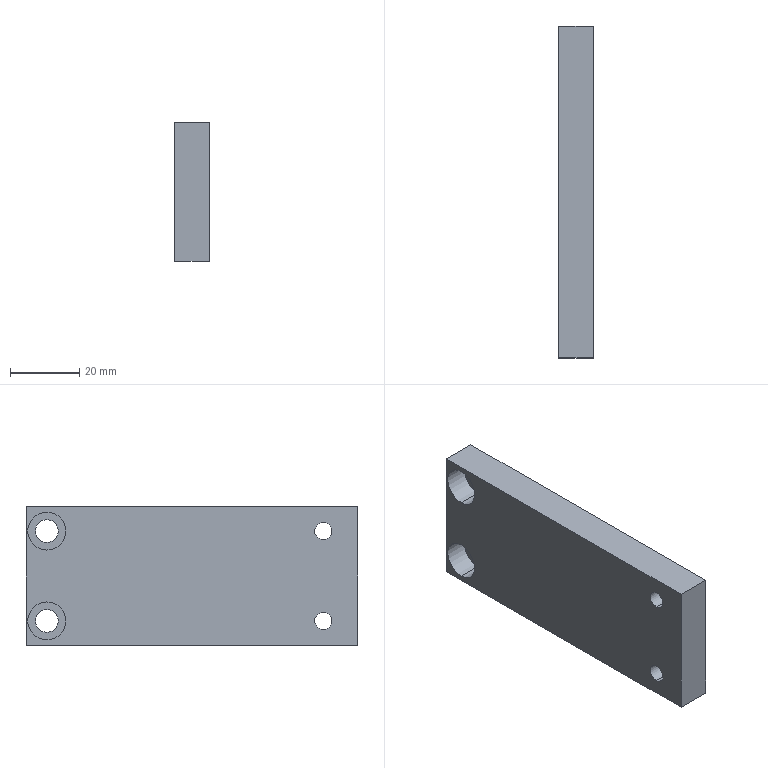Component | SolidWorks | SL021-102-4073.SL4PRT-1 | 1 solid | 20 faces | box 10 x 96 x 40 mm | volume 36496 mm3 | cylinder 12 | plane 8 | commonest cylinder face diameters 11 x4 6.6 x4 5 x4 | material AL6061
build123d program:
from build123d import *

# Parameters (mm, degrees)
SKETCH1_W                                          = 40
SKETCH1_H                                          = 96
BOSS_EXTRUDE1_DEPTH                                = 5
M6_TAPPED_HOLE1_D                                  = 5
HOLE_SIZE_ACCORDING_TO_TYPE_1_OF_HEXAG_D           = 6.6
HOLE_SIZE_ACCORDING_TO_TYPE_1_OF_HEXAG_CBORE_D     = 11
HOLE_SIZE_ACCORDING_TO_TYPE_1_OF_HEXAG_CBORE_DEPTH = 6.8


with BuildPart() as part:
    # Sketch1 → Boss-Extrude1 (new, symmetric)
    with BuildSketch(Plane.XY):
        Rectangle(SKETCH1_W, SKETCH1_H)
    extrude(amount=BOSS_EXTRUDE1_DEPTH, both=True)

    # M6 Tapped Hole1 (through all)
    with Locations(Plane.XY.offset(5)):
        with Locations((-13, -38), (13, -38)):
            Hole(M6_TAPPED_HOLE1_D / 2)

    # Hole Size _According to_ Type 1 of Hexag (through all)
    with Locations(Plane.XY.offset(5)):
        with Locations((-13, 42), (13, 42)):
            CounterBoreHole(HOLE_SIZE_ACCORDING_TO_TYPE_1_OF_HEXAG_D / 2, HOLE_SIZE_ACCORDING_TO_TYPE_1_OF_HEXAG_CBORE_D / 2, HOLE_SIZE_ACCORDING_TO_TYPE_1_OF_HEXAG_CBORE_DEPTH)


solid = part.part

# Placed as in the assembly
solid = solid.moved(Location((30.837, 137.501, -198.378), (0, -90, 0)))
STEP:
#1=COLOUR_RGB('',0.7922,0.8196,0.9333);
#2=FILL_AREA_STYLE_COLOUR('',#1);
#3=FILL_AREA_STYLE('',(#2));
#4=SURFACE_STYLE_FILL_AREA(#3);
#5=SURFACE_SIDE_STYLE('',(#4));
#6=SURFACE_STYLE_USAGE(.BOTH.,#5);
#7=PRESENTATION_STYLE_ASSIGNMENT((#6));
#8=CARTESIAN_POINT('',(1.285,7.067,-8.539));
#9=VERTEX_POINT('',#8);
#10=CARTESIAN_POINT('',(1.285,7.067,-8.105));
#11=VERTEX_POINT('',#10);
#12=CARTESIAN_POINT('',(1.285,7.067,-8.322));
#13=DIRECTION('',(-1.,0.,-0.));
#14=DIRECTION('',(0.,0.,1.));
#15=AXIS2_PLACEMENT_3D('',#12,#13,#14);
#16=CIRCLE('',#15,0.2165);
#17=EDGE_CURVE('',#9,#11,#16,.T.);
#18=ORIENTED_EDGE('',*,*,#17,.F.);
#19=CARTESIAN_POINT('',(1.017,7.067,-8.539));
#20=VERTEX_POINT('',#19);
#21=CARTESIAN_POINT('',(1.017,7.067,-8.539));
#22=DIRECTION('',(-1.,0.,-0.));
#23=VECTOR('',#22,39.37);
#24=LINE('',#21,#23);
#25=EDGE_CURVE('',#9,#20,#24,.T.);
#26=ORIENTED_EDGE('',*,*,#25,.T.);
#27=CARTESIAN_POINT('',(1.017,7.067,-8.105));
#28=VERTEX_POINT('',#27);
#29=CARTESIAN_POINT('',(1.017,7.067,-8.322));
#30=DIRECTION('',(-1.,0.,-0.));
#31=DIRECTION('',(0.,0.,1.));
#32=AXIS2_PLACEMENT_3D('',#29,#30,#31);
#33=CIRCLE('',#32,0.2165);
#34=EDGE_CURVE('',#20,#28,#33,.T.);
#35=ORIENTED_EDGE('',*,*,#34,.T.);
#36=CARTESIAN_POINT('',(1.017,7.067,-8.105));
#37=DIRECTION('',(-1.,0.,-0.));
#38=VECTOR('',#37,39.37);
#39=LINE('',#36,#38);
#40=EDGE_CURVE('',#11,#28,#39,.T.);
#41=ORIENTED_EDGE('',*,*,#40,.F.);
#42=EDGE_LOOP('',(#18,#26,#35,#41));
#43=FACE_OUTER_BOUND('',#42,.T.);
#44=CARTESIAN_POINT('',(1.017,7.067,-8.322));
#45=DIRECTION('',(-1.,0.,-0.));
#46=DIRECTION('',(0.,0.,1.));
#47=AXIS2_PLACEMENT_3D('',#44,#45,#46);
#48=CYLINDRICAL_SURFACE('',#47,0.2165);
#49=ADVANCED_FACE('',(#43),#48,.F.);
#50=CARTESIAN_POINT('',(1.411,7.067,-8.452));
#51=VERTEX_POINT('',#50);
#52=CARTESIAN_POINT('',(1.411,7.067,-8.192));
#53=VERTEX_POINT('',#52);
#54=CARTESIAN_POINT('',(1.411,7.067,-8.322));
#55=DIRECTION('',(-1.,0.,-0.));
#56=DIRECTION('',(0.,0.,1.));
#57=AXIS2_PLACEMENT_3D('',#54,#55,#56);
#58=CIRCLE('',#57,0.1299);
#59=EDGE_CURVE('',#51,#53,#58,.T.);
#60=ORIENTED_EDGE('',*,*,#59,.F.);
#61=CARTESIAN_POINT('',(1.285,7.067,-8.452));
#62=VERTEX_POINT('',#61);
#63=CARTESIAN_POINT('',(1.017,7.067,-8.452));
#64=DIRECTION('',(-1.,0.,-0.));
#65=VECTOR('',#64,39.37);
#66=LINE('',#63,#65);
#67=EDGE_CURVE('',#51,#62,#66,.T.);
#68=ORIENTED_EDGE('',*,*,#67,.T.);
#69=CARTESIAN_POINT('',(1.285,7.067,-8.192));
#70=VERTEX_POINT('',#69);
#71=CARTESIAN_POINT('',(1.285,7.067,-8.322));
#72=DIRECTION('',(-1.,0.,-0.));
#73=DIRECTION('',(0.,0.,1.));
#74=AXIS2_PLACEMENT_3D('',#71,#72,#73);
#75=CIRCLE('',#74,0.1299);
#76=EDGE_CURVE('',#62,#70,#75,.T.);
#77=ORIENTED_EDGE('',*,*,#76,.T.);
#78=CARTESIAN_POINT('',(1.017,7.067,-8.192));
#79=DIRECTION('',(-1.,0.,-0.));
#80=VECTOR('',#79,39.37);
#81=LINE('',#78,#80);
#82=EDGE_CURVE('',#53,#70,#81,.T.);
#83=ORIENTED_EDGE('',*,*,#82,.F.);
#84=EDGE_LOOP('',(#60,#68,#77,#83));
#85=FACE_OUTER_BOUND('',#84,.T.);
#86=CARTESIAN_POINT('',(1.017,7.067,-8.322));
#87=DIRECTION('',(-1.,0.,-0.));
#88=DIRECTION('',(0.,0.,1.));
#89=AXIS2_PLACEMENT_3D('',#86,#87,#88);
#90=CYLINDRICAL_SURFACE('',#89,0.1299);
#91=ADVANCED_FACE('',(#85),#90,.F.);
#92=CARTESIAN_POINT('',(1.285,7.067,-7.515));
#93=VERTEX_POINT('',#92);
#94=CARTESIAN_POINT('',(1.285,7.067,-7.082));
#95=VERTEX_POINT('',#94);
#96=CARTESIAN_POINT('',(1.285,7.067,-7.298));
#97=DIRECTION('',(-1.,0.,-0.));
#98=DIRECTION('',(0.,0.,1.));
#99=AXIS2_PLACEMENT_3D('',#96,#97,#98);
#100=CIRCLE('',#99,0.2165);
#101=EDGE_CURVE('',#93,#95,#100,.T.);
#102=ORIENTED_EDGE('',*,*,#101,.F.);
#103=CARTESIAN_POINT('',(1.017,7.067,-7.515));
#104=VERTEX_POINT('',#103);
#105=CARTESIAN_POINT('',(1.017,7.067,-7.515));
#106=DIRECTION('',(-1.,0.,-0.));
#107=VECTOR('',#106,39.37);
#108=LINE('',#105,#107);
#109=EDGE_CURVE('',#93,#104,#108,.T.);
#110=ORIENTED_EDGE('',*,*,#109,.T.);
#111=CARTESIAN_POINT('',(1.017,7.067,-7.082));
#112=VERTEX_POINT('',#111);
#113=CARTESIAN_POINT('',(1.017,7.067,-7.298));
#114=DIRECTION('',(-1.,0.,-0.));
#115=DIRECTION('',(0.,0.,1.));
#116=AXIS2_PLACEMENT_3D('',#113,#114,#115);
#117=CIRCLE('',#116,0.2165);
#118=EDGE_CURVE('',#104,#112,#117,.T.);
#119=ORIENTED_EDGE('',*,*,#118,.T.);
#120=CARTESIAN_POINT('',(1.017,7.067,-7.082));
#121=DIRECTION('',(-1.,0.,-0.));
#122=VECTOR('',#121,39.37);
#123=LINE('',#120,#122);
#124=EDGE_CURVE('',#95,#112,#123,.T.);
#125=ORIENTED_EDGE('',*,*,#124,.F.);
#126=EDGE_LOOP('',(#102,#110,#119,#125));
#127=FACE_OUTER_BOUND('',#126,.T.);
#128=CARTESIAN_POINT('',(1.017,7.067,-7.298));
#129=DIRECTION('',(-1.,0.,-0.));
#130=DIRECTION('',(0.,0.,1.));
#131=AXIS2_PLACEMENT_3D('',#128,#129,#130);
#132=CYLINDRICAL_SURFACE('',#131,0.2165);
#133=ADVANCED_FACE('',(#127),#132,.F.);
#134=CARTESIAN_POINT('',(1.411,7.067,-7.428));
#135=VERTEX_POINT('',#134);
#136=CARTESIAN_POINT('',(1.411,7.067,-7.168));
#137=VERTEX_POINT('',#136);
#138=CARTESIAN_POINT('',(1.411,7.067,-7.298));
#139=DIRECTION('',(-1.,0.,-0.));
#140=DIRECTION('',(0.,0.,1.));
#141=AXIS2_PLACEMENT_3D('',#138,#139,#140);
#142=CIRCLE('',#141,0.1299);
#143=EDGE_CURVE('',#135,#137,#142,.T.);
#144=ORIENTED_EDGE('',*,*,#143,.F.);
#145=CARTESIAN_POINT('',(1.285,7.067,-7.428));
#146=VERTEX_POINT('',#145);
#147=CARTESIAN_POINT('',(1.017,7.067,-7.428));
#148=DIRECTION('',(-1.,0.,-0.));
#149=VECTOR('',#148,39.37);
#150=LINE('',#147,#149);
#151=EDGE_CURVE('',#135,#146,#150,.T.);
#152=ORIENTED_EDGE('',*,*,#151,.T.);
#153=CARTESIAN_POINT('',(1.285,7.067,-7.168));
#154=VERTEX_POINT('',#153);
#155=CARTESIAN_POINT('',(1.285,7.067,-7.298));
#156=DIRECTION('',(-1.,0.,-0.));
#157=DIRECTION('',(0.,0.,1.));
#158=AXIS2_PLACEMENT_3D('',#155,#156,#157);
#159=CIRCLE('',#158,0.1299);
#160=EDGE_CURVE('',#146,#154,#159,.T.);
#161=ORIENTED_EDGE('',*,*,#160,.T.);
#162=CARTESIAN_POINT('',(1.017,7.067,-7.168));
#163=DIRECTION('',(-1.,0.,-0.));
#164=VECTOR('',#163,39.37);
#165=LINE('',#162,#164);
#166=EDGE_CURVE('',#137,#154,#165,.T.);
#167=ORIENTED_EDGE('',*,*,#166,.F.);
#168=EDGE_LOOP('',(#144,#152,#161,#167));
#169=FACE_OUTER_BOUND('',#168,.T.);
#170=CARTESIAN_POINT('',(1.017,7.067,-7.298));
#171=DIRECTION('',(-1.,0.,-0.));
#172=DIRECTION('',(0.,0.,1.));
#173=AXIS2_PLACEMENT_3D('',#170,#171,#172);
#174=CYLINDRICAL_SURFACE('',#173,0.1299);
#175=ADVANCED_FACE('',(#169),#174,.F.);
#176=CARTESIAN_POINT('',(1.411,3.917,-8.42));
#177=VERTEX_POINT('',#176);
#178=CARTESIAN_POINT('',(1.411,3.917,-8.224));
#179=VERTEX_POINT('',#178);
#180=CARTESIAN_POINT('',(1.411,3.917,-8.322));
#181=DIRECTION('',(-1.,0.,-0.));
#182=DIRECTION('',(0.,0.,1.));
#183=AXIS2_PLACEMENT_3D('',#180,#181,#182);
#184=CIRCLE('',#183,0.09843);
#185=EDGE_CURVE('',#177,#179,#184,.T.);
#186=ORIENTED_EDGE('',*,*,#185,.F.);
#187=CARTESIAN_POINT('',(1.017,3.917,-8.42));
#188=VERTEX_POINT('',#187);
#189=CARTESIAN_POINT('',(1.017,3.917,-8.42));
#190=DIRECTION('',(-1.,0.,-0.));
#191=VECTOR('',#190,39.37);
#192=LINE('',#189,#191);
#193=EDGE_CURVE('',#177,#188,#192,.T.);
#194=ORIENTED_EDGE('',*,*,#193,.T.);
#195=CARTESIAN_POINT('',(1.017,3.917,-8.224));
#196=VERTEX_POINT('',#195);
#197=CARTESIAN_POINT('',(1.017,3.917,-8.322));
#198=DIRECTION('',(-1.,0.,-0.));
#199=DIRECTION('',(0.,0.,1.));
#200=AXIS2_PLACEMENT_3D('',#197,#198,#199);
#201=CIRCLE('',#200,0.09843);
#202=EDGE_CURVE('',#188,#196,#201,.T.);
#203=ORIENTED_EDGE('',*,*,#202,.T.);
#204=CARTESIAN_POINT('',(1.017,3.917,-8.224));
#205=DIRECTION('',(-1.,0.,-0.));
#206=VECTOR('',#205,39.37);
#207=LINE('',#204,#206);
#208=EDGE_CURVE('',#179,#196,#207,.T.);
#209=ORIENTED_EDGE('',*,*,#208,.F.);
#210=EDGE_LOOP('',(#186,#194,#203,#209));
#211=FACE_OUTER_BOUND('',#210,.T.);
#212=CARTESIAN_POINT('',(1.017,3.917,-8.322));
#213=DIRECTION('',(-1.,0.,-0.));
#214=DIRECTION('',(0.,0.,1.));
#215=AXIS2_PLACEMENT_3D('',#212,#213,#214);
#216=CYLINDRICAL_SURFACE('',#215,0.09843);
#217=ADVANCED_FACE('',(#211),#216,.F.);
#218=CARTESIAN_POINT('',(1.411,3.917,-7.397));
#219=VERTEX_POINT('',#218);
#220=CARTESIAN_POINT('',(1.411,3.917,-7.2));
#221=VERTEX_POINT('',#220);
#222=CARTESIAN_POINT('',(1.411,3.917,-7.298));
#223=DIRECTION('',(-1.,0.,-0.));
#224=DIRECTION('',(0.,0.,1.));
#225=AXIS2_PLACEMENT_3D('',#222,#223,#224);
#226=CIRCLE('',#225,0.09843);
#227=EDGE_CURVE('',#219,#221,#226,.T.);
#228=ORIENTED_EDGE('',*,*,#227,.F.);
#229=CARTESIAN_POINT('',(1.017,3.917,-7.397));
#230=VERTEX_POINT('',#229);
#231=CARTESIAN_POINT('',(1.017,3.917,-7.397));
#232=DIRECTION('',(-1.,0.,-0.));
#233=VECTOR('',#232,39.37);
#234=LINE('',#231,#233);
#235=EDGE_CURVE('',#219,#230,#234,.T.);
#236=ORIENTED_EDGE('',*,*,#235,.T.);
#237=CARTESIAN_POINT('',(1.017,3.917,-7.2));
#238=VERTEX_POINT('',#237);
#239=CARTESIAN_POINT('',(1.017,3.917,-7.298));
#240=DIRECTION('',(-1.,0.,-0.));
#241=DIRECTION('',(0.,0.,1.));
#242=AXIS2_PLACEMENT_3D('',#239,#240,#241);
#243=CIRCLE('',#242,0.09843);
#244=EDGE_CURVE('',#230,#238,#243,.T.);
#245=ORIENTED_EDGE('',*,*,#244,.T.);
#246=CARTESIAN_POINT('',(1.017,3.917,-7.2));
#247=DIRECTION('',(-1.,0.,-0.));
#248=VECTOR('',#247,39.37);
#249=LINE('',#246,#248);
#250=EDGE_CURVE('',#221,#238,#249,.T.);
#251=ORIENTED_EDGE('',*,*,#250,.F.);
#252=EDGE_LOOP('',(#228,#236,#245,#251));
#253=FACE_OUTER_BOUND('',#252,.T.);
#254=CARTESIAN_POINT('',(1.017,3.917,-7.298));
#255=DIRECTION('',(-1.,0.,-0.));
#256=DIRECTION('',(0.,0.,1.));
#257=AXIS2_PLACEMENT_3D('',#254,#255,#256);
#258=CYLINDRICAL_SURFACE('',#257,0.09843);
#259=ADVANCED_FACE('',(#253),#258,.F.);
#260=CARTESIAN_POINT('',(1.411,7.067,-8.322));
#261=DIRECTION('',(-1.,0.,-0.));
#262=DIRECTION('',(0.,0.,1.));
#263=AXIS2_PLACEMENT_3D('',#260,#261,#262);
#264=CIRCLE('',#263,0.1299);
#265=EDGE_CURVE('',#53,#51,#264,.T.);
#266=ORIENTED_EDGE('',*,*,#265,.T.);
#267=ORIENTED_EDGE('',*,*,#59,.T.);
#268=EDGE_LOOP('',(#266,#267));
#269=FACE_BOUND('',#268,.T.);
#270=CARTESIAN_POINT('',(1.411,7.067,-7.298));
#271=DIRECTION('',(-1.,0.,-0.));
#272=DIRECTION('',(0.,0.,1.));
#273=AXIS2_PLACEMENT_3D('',#270,#271,#272);
#274=CIRCLE('',#273,0.1299);
#275=EDGE_CURVE('',#137,#135,#274,.T.);
#276=ORIENTED_EDGE('',*,*,#275,.T.);
#277=ORIENTED_EDGE('',*,*,#143,.T.);
#278=EDGE_LOOP('',(#276,#277));
#279=FACE_BOUND('',#278,.T.);
#280=CARTESIAN_POINT('',(1.411,3.524,-7.023));
#281=VERTEX_POINT('',#280);
#282=CARTESIAN_POINT('',(1.411,7.303,-7.023));
#283=VERTEX_POINT('',#282);
#284=CARTESIAN_POINT('',(1.411,3.524,-7.023));
#285=DIRECTION('',(0.,1.,0.));
#286=VECTOR('',#285,39.37);
#287=LINE('',#284,#286);
#288=EDGE_CURVE('',#281,#283,#287,.T.);
#289=ORIENTED_EDGE('',*,*,#288,.F.);
#290=CARTESIAN_POINT('',(1.411,3.524,-8.598));
#291=VERTEX_POINT('',#290);
#292=CARTESIAN_POINT('',(1.411,3.524,-8.598));
#293=DIRECTION('',(-0.,-0.,1.));
#294=VECTOR('',#293,39.37);
#295=LINE('',#292,#294);
#296=EDGE_CURVE('',#291,#281,#295,.T.);
#297=ORIENTED_EDGE('',*,*,#296,.F.);
#298=CARTESIAN_POINT('',(1.411,7.303,-8.598));
#299=VERTEX_POINT('',#298);
#300=CARTESIAN_POINT('',(1.411,3.524,-8.598));
#301=DIRECTION('',(-0.,-1.,-0.));
#302=VECTOR('',#301,39.37);
#303=LINE('',#300,#302);
#304=EDGE_CURVE('',#299,#291,#303,.T.);
#305=ORIENTED_EDGE('',*,*,#304,.F.);
#306=CARTESIAN_POINT('',(1.411,7.303,-8.598));
#307=DIRECTION('',(0.,0.,-1.));
#308=VECTOR('',#307,39.37);
#309=LINE('',#306,#308);
#310=EDGE_CURVE('',#283,#299,#309,.T.);
#311=ORIENTED_EDGE('',*,*,#310,.F.);
#312=EDGE_LOOP('',(#289,#297,#305,#311));
#313=FACE_OUTER_BOUND('',#312,.T.);
#314=CARTESIAN_POINT('',(1.411,3.917,-7.298));
#315=DIRECTION('',(-1.,0.,-0.));
#316=DIRECTION('',(0.,0.,1.));
#317=AXIS2_PLACEMENT_3D('',#314,#315,#316);
#318=CIRCLE('',#317,0.09843);
#319=EDGE_CURVE('',#221,#219,#318,.T.);
#320=ORIENTED_EDGE('',*,*,#319,.T.);
#321=ORIENTED_EDGE('',*,*,#227,.T.);
#322=EDGE_LOOP('',(#320,#321));
#323=FACE_BOUND('',#322,.T.);
#324=CARTESIAN_POINT('',(1.411,3.917,-8.322));
#325=DIRECTION('',(-1.,0.,-0.));
#326=DIRECTION('',(0.,0.,1.));
#327=AXIS2_PLACEMENT_3D('',#324,#325,#326);
#328=CIRCLE('',#327,0.09843);
#329=EDGE_CURVE('',#179,#177,#328,.T.);
#330=ORIENTED_EDGE('',*,*,#329,.T.);
#331=ORIENTED_EDGE('',*,*,#185,.T.);
#332=EDGE_LOOP('',(#330,#331));
#333=FACE_BOUND('',#332,.T.);
#334=CARTESIAN_POINT('',(1.411,5.413,-7.81));
#335=DIRECTION('',(1.,-0.,0.));
#336=DIRECTION('',(0.,0.,-1.));
#337=AXIS2_PLACEMENT_3D('',#334,#335,#336);
#338=PLANE('',#337);
#339=ADVANCED_FACE('',(#269,#279,#313,#323,#333),#338,.T.);
#340=ORIENTED_EDGE('',*,*,#288,.T.);
#341=CARTESIAN_POINT('',(1.017,7.303,-7.023));
#342=VERTEX_POINT('',#341);
#343=CARTESIAN_POINT('',(1.017,7.303,-7.023));
#344=DIRECTION('',(1.,-0.,0.));
#345=VECTOR('',#344,39.37);
#346=LINE('',#343,#345);
#347=EDGE_CURVE('',#342,#283,#346,.T.);
#348=ORIENTED_EDGE('',*,*,#347,.F.);
#349=CARTESIAN_POINT('',(1.017,3.524,-7.023));
#350=VERTEX_POINT('',#349);
#351=CARTESIAN_POINT('',(1.017,3.524,-7.023));
#352=DIRECTION('',(0.,1.,0.));
#353=VECTOR('',#352,39.37);
#354=LINE('',#351,#353);
#355=EDGE_CURVE('',#350,#342,#354,.T.);
#356=ORIENTED_EDGE('',*,*,#355,.F.);
#357=CARTESIAN_POINT('',(1.017,3.524,-7.023));
#358=DIRECTION('',(1.,-0.,0.));
#359=VECTOR('',#358,39.37);
#360=LINE('',#357,#359);
#361=EDGE_CURVE('',#350,#281,#360,.T.);
#362=ORIENTED_EDGE('',*,*,#361,.T.);
#363=EDGE_LOOP('',(#340,#348,#356,#362));
#364=FACE_OUTER_BOUND('',#363,.T.);
#365=CARTESIAN_POINT('',(1.017,3.524,-7.023));
#366=DIRECTION('',(0.,0.,-1.));
#367=DIRECTION('',(-1.,0.,-0.));
#368=AXIS2_PLACEMENT_3D('',#365,#366,#367);
#369=PLANE('',#368);
#370=ADVANCED_FACE('',(#364),#369,.F.);
#371=ORIENTED_EDGE('',*,*,#310,.T.);
#372=CARTESIAN_POINT('',(1.017,7.303,-8.598));
#373=VERTEX_POINT('',#372);
#374=CARTESIAN_POINT('',(1.017,7.303,-8.598));
#375=DIRECTION('',(1.,-0.,0.));
#376=VECTOR('',#375,39.37);
#377=LINE('',#374,#376);
#378=EDGE_CURVE('',#373,#299,#377,.T.);
#379=ORIENTED_EDGE('',*,*,#378,.F.);
#380=CARTESIAN_POINT('',(1.017,7.303,-8.598));
#381=DIRECTION('',(0.,0.,-1.));
#382=VECTOR('',#381,39.37);
#383=LINE('',#380,#382);
#384=EDGE_CURVE('',#342,#373,#383,.T.);
#385=ORIENTED_EDGE('',*,*,#384,.F.);
#386=ORIENTED_EDGE('',*,*,#347,.T.);
#387=EDGE_LOOP('',(#371,#379,#385,#386));
#388=FACE_OUTER_BOUND('',#387,.T.);
#389=CARTESIAN_POINT('',(1.017,7.303,-8.598));
#390=DIRECTION('',(-0.,-1.,-0.));
#391=DIRECTION('',(1.,-0.,0.));
#392=AXIS2_PLACEMENT_3D('',#389,#390,#391);
#393=PLANE('',#392);
#394=ADVANCED_FACE('',(#388),#393,.F.);
#395=ORIENTED_EDGE('',*,*,#304,.T.);
#396=CARTESIAN_POINT('',(1.017,3.524,-8.598));
#397=VERTEX_POINT('',#396);
#398=CARTESIAN_POINT('',(1.017,3.524,-8.598));
#399=DIRECTION('',(1.,-0.,0.));
#400=VECTOR('',#399,39.37);
#401=LINE('',#398,#400);
#402=EDGE_CURVE('',#397,#291,#401,.T.);
#403=ORIENTED_EDGE('',*,*,#402,.F.);
#404=CARTESIAN_POINT('',(1.017,3.524,-8.598));
#405=DIRECTION('',(-0.,-1.,-0.));
#406=VECTOR('',#405,39.37);
#407=LINE('',#404,#406);
#408=EDGE_CURVE('',#373,#397,#407,.T.);
#409=ORIENTED_EDGE('',*,*,#408,.F.);
#410=ORIENTED_EDGE('',*,*,#378,.T.);
#411=EDGE_LOOP('',(#395,#403,#409,#410));
#412=FACE_OUTER_BOUND('',#411,.T.);
#413=CARTESIAN_POINT('',(1.017,3.524,-8.598));
#414=DIRECTION('',(-0.,-0.,1.));
#415=DIRECTION('',(1.,-0.,0.));
#416=AXIS2_PLACEMENT_3D('',#413,#414,#415);
#417=PLANE('',#416);
#418=ADVANCED_FACE('',(#412),#417,.F.);
#419=ORIENTED_EDGE('',*,*,#296,.T.);
#420=ORIENTED_EDGE('',*,*,#361,.F.);
#421=CARTESIAN_POINT('',(1.017,3.524,-8.598));
#422=DIRECTION('',(-0.,-0.,1.));
#423=VECTOR('',#422,39.37);
#424=LINE('',#421,#423);
#425=EDGE_CURVE('',#397,#350,#424,.T.);
#426=ORIENTED_EDGE('',*,*,#425,.F.);
#427=ORIENTED_EDGE('',*,*,#402,.T.);
#428=EDGE_LOOP('',(#419,#420,#426,#427));
#429=FACE_OUTER_BOUND('',#428,.T.);
#430=CARTESIAN_POINT('',(1.017,3.524,-8.598));
#431=DIRECTION('',(0.,1.,0.));
#432=DIRECTION('',(-1.,0.,-0.));
#433=AXIS2_PLACEMENT_3D('',#430,#431,#432);
#434=PLANE('',#433);
#435=ADVANCED_FACE('',(#429),#434,.F.);
#436=CARTESIAN_POINT('',(1.017,7.067,-8.322));
#437=DIRECTION('',(-1.,0.,-0.));
#438=DIRECTION('',(0.,0.,1.));
#439=AXIS2_PLACEMENT_3D('',#436,#437,#438);
#440=CIRCLE('',#439,0.2165);
#441=EDGE_CURVE('',#28,#20,#440,.T.);
#442=ORIENTED_EDGE('',*,*,#441,.F.);
#443=ORIENTED_EDGE('',*,*,#34,.F.);
#444=EDGE_LOOP('',(#442,#443));
#445=FACE_BOUND('',#444,.T.);
#446=CARTESIAN_POINT('',(1.017,7.067,-7.298));
#447=DIRECTION('',(-1.,0.,-0.));
#448=DIRECTION('',(0.,0.,1.));
#449=AXIS2_PLACEMENT_3D('',#446,#447,#448);
#450=CIRCLE('',#449,0.2165);
#451=EDGE_CURVE('',#112,#104,#450,.T.);
#452=ORIENTED_EDGE('',*,*,#451,.F.);
#453=ORIENTED_EDGE('',*,*,#118,.F.);
#454=EDGE_LOOP('',(#452,#453));
#455=FACE_BOUND('',#454,.T.);
#456=CARTESIAN_POINT('',(1.017,3.917,-8.322));
#457=DIRECTION('',(-1.,0.,-0.));
#458=DIRECTION('',(0.,0.,1.));
#459=AXIS2_PLACEMENT_3D('',#456,#457,#458);
#460=CIRCLE('',#459,0.09843);
#461=EDGE_CURVE('',#196,#188,#460,.T.);
#462=ORIENTED_EDGE('',*,*,#461,.F.);
#463=ORIENTED_EDGE('',*,*,#202,.F.);
#464=EDGE_LOOP('',(#462,#463));
#465=FACE_BOUND('',#464,.T.);
#466=CARTESIAN_POINT('',(1.017,3.917,-7.298));
#467=DIRECTION('',(-1.,0.,-0.));
#468=DIRECTION('',(0.,0.,1.));
#469=AXIS2_PLACEMENT_3D('',#466,#467,#468);
#470=CIRCLE('',#469,0.09843);
#471=EDGE_CURVE('',#238,#230,#470,.T.);
#472=ORIENTED_EDGE('',*,*,#471,.F.);
#473=ORIENTED_EDGE('',*,*,#244,.F.);
#474=EDGE_LOOP('',(#472,#473));
#475=FACE_BOUND('',#474,.T.);
#476=ORIENTED_EDGE('',*,*,#355,.T.);
#477=ORIENTED_EDGE('',*,*,#384,.T.);
#478=ORIENTED_EDGE('',*,*,#408,.T.);
#479=ORIENTED_EDGE('',*,*,#425,.T.);
#480=EDGE_LOOP('',(#476,#477,#478,#479));
#481=FACE_OUTER_BOUND('',#480,.T.);
#482=CARTESIAN_POINT('',(1.017,5.413,-7.81));
#483=DIRECTION('',(1.,-0.,0.));
#484=DIRECTION('',(0.,0.,-1.));
#485=AXIS2_PLACEMENT_3D('',#482,#483,#484);
#486=PLANE('',#485);
#487=ADVANCED_FACE('',(#445,#455,#465,#475,#481),#486,.F.);
#488=ORIENTED_EDGE('',*,*,#235,.F.);
#489=ORIENTED_EDGE('',*,*,#319,.F.);
#490=ORIENTED_EDGE('',*,*,#250,.T.);
#491=ORIENTED_EDGE('',*,*,#471,.T.);
#492=EDGE_LOOP('',(#488,#489,#490,#491));
#493=FACE_OUTER_BOUND('',#492,.T.);
#494=CARTESIAN_POINT('',(1.017,3.917,-7.298));
#495=DIRECTION('',(-1.,0.,-0.));
#496=DIRECTION('',(0.,0.,1.));
#497=AXIS2_PLACEMENT_3D('',#494,#495,#496);
#498=CYLINDRICAL_SURFACE('',#497,0.09843);
#499=ADVANCED_FACE('',(#493),#498,.F.);
#500=ORIENTED_EDGE('',*,*,#193,.F.);
#501=ORIENTED_EDGE('',*,*,#329,.F.);
#502=ORIENTED_EDGE('',*,*,#208,.T.);
#503=ORIENTED_EDGE('',*,*,#461,.T.);
#504=EDGE_LOOP('',(#500,#501,#502,#503));
#505=FACE_OUTER_BOUND('',#504,.T.);
#506=CARTESIAN_POINT('',(1.017,3.917,-8.322));
#507=DIRECTION('',(-1.,0.,-0.));
#508=DIRECTION('',(0.,0.,1.));
#509=AXIS2_PLACEMENT_3D('',#506,#507,#508);
#510=CYLINDRICAL_SURFACE('',#509,0.09843);
#511=ADVANCED_FACE('',(#505),#510,.F.);
#512=ORIENTED_EDGE('',*,*,#151,.F.);
#513=ORIENTED_EDGE('',*,*,#275,.F.);
#514=ORIENTED_EDGE('',*,*,#166,.T.);
#515=CARTESIAN_POINT('',(1.285,7.067,-7.298));
#516=DIRECTION('',(-1.,0.,-0.));
#517=DIRECTION('',(0.,0.,1.));
#518=AXIS2_PLACEMENT_3D('',#515,#516,#517);
#519=CIRCLE('',#518,0.1299);
#520=EDGE_CURVE('',#154,#146,#519,.T.);
#521=ORIENTED_EDGE('',*,*,#520,.T.);
#522=EDGE_LOOP('',(#512,#513,#514,#521));
#523=FACE_OUTER_BOUND('',#522,.T.);
#524=CARTESIAN_POINT('',(1.017,7.067,-7.298));
#525=DIRECTION('',(-1.,0.,-0.));
#526=DIRECTION('',(0.,0.,1.));
#527=AXIS2_PLACEMENT_3D('',#524,#525,#526);
#528=CYLINDRICAL_SURFACE('',#527,0.1299);
#529=ADVANCED_FACE('',(#523),#528,.F.);
#530=ORIENTED_EDGE('',*,*,#520,.F.);
#531=ORIENTED_EDGE('',*,*,#160,.F.);
#532=EDGE_LOOP('',(#530,#531));
#533=FACE_BOUND('',#532,.T.);
#534=CARTESIAN_POINT('',(1.285,7.067,-7.298));
#535=DIRECTION('',(-1.,0.,-0.));
#536=DIRECTION('',(0.,0.,1.));
#537=AXIS2_PLACEMENT_3D('',#534,#535,#536);
#538=CIRCLE('',#537,0.2165);
#539=EDGE_CURVE('',#95,#93,#538,.T.);
#540=ORIENTED_EDGE('',*,*,#539,.T.);
#541=ORIENTED_EDGE('',*,*,#101,.T.);
#542=EDGE_LOOP('',(#540,#541));
#543=FACE_OUTER_BOUND('',#542,.T.);
#544=CARTESIAN_POINT('',(1.285,7.067,-7.168));
#545=DIRECTION('',(1.,-0.,0.));
#546=DIRECTION('',(0.,0.,-1.));
#547=AXIS2_PLACEMENT_3D('',#544,#545,#546);
#548=PLANE('',#547);
#549=ADVANCED_FACE('',(#533,#543),#548,.F.);
#550=ORIENTED_EDGE('',*,*,#109,.F.);
#551=ORIENTED_EDGE('',*,*,#539,.F.);
#552=ORIENTED_EDGE('',*,*,#124,.T.);
#553=ORIENTED_EDGE('',*,*,#451,.T.);
#554=EDGE_LOOP('',(#550,#551,#552,#553));
#555=FACE_OUTER_BOUND('',#554,.T.);
#556=CARTESIAN_POINT('',(1.017,7.067,-7.298));
#557=DIRECTION('',(-1.,0.,-0.));
#558=DIRECTION('',(0.,0.,1.));
#559=AXIS2_PLACEMENT_3D('',#556,#557,#558);
#560=CYLINDRICAL_SURFACE('',#559,0.2165);
#561=ADVANCED_FACE('',(#555),#560,.F.);
#562=ORIENTED_EDGE('',*,*,#67,.F.);
#563=ORIENTED_EDGE('',*,*,#265,.F.);
#564=ORIENTED_EDGE('',*,*,#82,.T.);
#565=CARTESIAN_POINT('',(1.285,7.067,-8.322));
#566=DIRECTION('',(-1.,0.,-0.));
#567=DIRECTION('',(0.,0.,1.));
#568=AXIS2_PLACEMENT_3D('',#565,#566,#567);
#569=CIRCLE('',#568,0.1299);
#570=EDGE_CURVE('',#70,#62,#569,.T.);
#571=ORIENTED_EDGE('',*,*,#570,.T.);
#572=EDGE_LOOP('',(#562,#563,#564,#571));
#573=FACE_OUTER_BOUND('',#572,.T.);
#574=CARTESIAN_POINT('',(1.017,7.067,-8.322));
#575=DIRECTION('',(-1.,0.,-0.));
#576=DIRECTION('',(0.,0.,1.));
#577=AXIS2_PLACEMENT_3D('',#574,#575,#576);
#578=CYLINDRICAL_SURFACE('',#577,0.1299);
#579=ADVANCED_FACE('',(#573),#578,.F.);
#580=ORIENTED_EDGE('',*,*,#570,.F.);
#581=ORIENTED_EDGE('',*,*,#76,.F.);
#582=EDGE_LOOP('',(#580,#581));
#583=FACE_BOUND('',#582,.T.);
#584=CARTESIAN_POINT('',(1.285,7.067,-8.322));
#585=DIRECTION('',(-1.,0.,-0.));
#586=DIRECTION('',(0.,0.,1.));
#587=AXIS2_PLACEMENT_3D('',#584,#585,#586);
#588=CIRCLE('',#587,0.2165);
#589=EDGE_CURVE('',#11,#9,#588,.T.);
#590=ORIENTED_EDGE('',*,*,#589,.T.);
#591=ORIENTED_EDGE('',*,*,#17,.T.);
#592=EDGE_LOOP('',(#590,#591));
#593=FACE_OUTER_BOUND('',#592,.T.);
#594=CARTESIAN_POINT('',(1.285,7.067,-8.192));
#595=DIRECTION('',(1.,-0.,0.));
#596=DIRECTION('',(0.,0.,-1.));
#597=AXIS2_PLACEMENT_3D('',#594,#595,#596);
#598=PLANE('',#597);
#599=ADVANCED_FACE('',(#583,#593),#598,.F.);
#600=ORIENTED_EDGE('',*,*,#25,.F.);
#601=ORIENTED_EDGE('',*,*,#589,.F.);
#602=ORIENTED_EDGE('',*,*,#40,.T.);
#603=ORIENTED_EDGE('',*,*,#441,.T.);
#604=EDGE_LOOP('',(#600,#601,#602,#603));
#605=FACE_OUTER_BOUND('',#604,.T.);
#606=CARTESIAN_POINT('',(1.017,7.067,-8.322));
#607=DIRECTION('',(-1.,0.,-0.));
#608=DIRECTION('',(0.,0.,1.));
#609=AXIS2_PLACEMENT_3D('',#606,#607,#608);
#610=CYLINDRICAL_SURFACE('',#609,0.2165);
#611=ADVANCED_FACE('',(#605),#610,.F.);
#612=CLOSED_SHELL('',(#49,#91,#133,#175,#217,#259,#339,#370,#394,#418,#435,#487,#499,#511,#529,#549,#561,#579,#599,#611));
#613=MANIFOLD_SOLID_BREP('',#612);
#614=STYLED_ITEM('',(#7),#613);
#615=PRESENTATION_LAYER_ASSIGNMENT('','',(#614));
#616=CARTESIAN_POINT('',(0.,0.,0.));
#617=DIRECTION('',(0.,0.,1.));
#618=DIRECTION('',(1.,0.,0.));
#619=AXIS2_PLACEMENT_3D('',#616,#617,#618);
#620=(LENGTH_UNIT()NAMED_UNIT(*)SI_UNIT($,.METRE.));
#621=LENGTH_MEASURE_WITH_UNIT(LENGTH_MEASURE(0.0254),#620);
#622=DIMENSIONAL_EXPONENTS(1.,0.,0.,0.,0.,0.,0.);
#623=(CONVERSION_BASED_UNIT('',#621)LENGTH_UNIT()NAMED_UNIT(#622));
#624=UNCERTAINTY_MEASURE_WITH_UNIT(LENGTH_MEASURE(0.00001),#623,'','');
#625=(NAMED_UNIT(*)PLANE_ANGLE_UNIT()SI_UNIT($,.RADIAN.));
#626=(NAMED_UNIT(*)SI_UNIT($,.STERADIAN.)SOLID_ANGLE_UNIT());
#627=(GEOMETRIC_REPRESENTATION_CONTEXT(3)GLOBAL_UNCERTAINTY_ASSIGNED_CONTEXT((#624))GLOBAL_UNIT_ASSIGNED_CONTEXT((#623,#625,#626))REPRESENTATION_CONTEXT('',''));
#628=ADVANCED_BREP_SHAPE_REPRESENTATION('',(#613,#619),#627);
#629=(LENGTH_UNIT()NAMED_UNIT(*)SI_UNIT($,.METRE.));
#630=LENGTH_MEASURE_WITH_UNIT(LENGTH_MEASURE(0.0254),#629);
#631=DIMENSIONAL_EXPONENTS(1.,0.,0.,0.,0.,0.,0.);
#632=(CONVERSION_BASED_UNIT('',#630)LENGTH_UNIT()NAMED_UNIT(#631));
#633=UNCERTAINTY_MEASURE_WITH_UNIT(LENGTH_MEASURE(0.00001),#632,'','');
#634=(NAMED_UNIT(*)PLANE_ANGLE_UNIT()SI_UNIT($,.RADIAN.));
#635=(NAMED_UNIT(*)SI_UNIT($,.STERADIAN.)SOLID_ANGLE_UNIT());
#636=(GEOMETRIC_REPRESENTATION_CONTEXT(3)GLOBAL_UNCERTAINTY_ASSIGNED_CONTEXT((#633))GLOBAL_UNIT_ASSIGNED_CONTEXT((#632,#634,#635))REPRESENTATION_CONTEXT('',''));
#637=MECHANICAL_DESIGN_GEOMETRIC_PRESENTATION_REPRESENTATION('',(#614),#636);